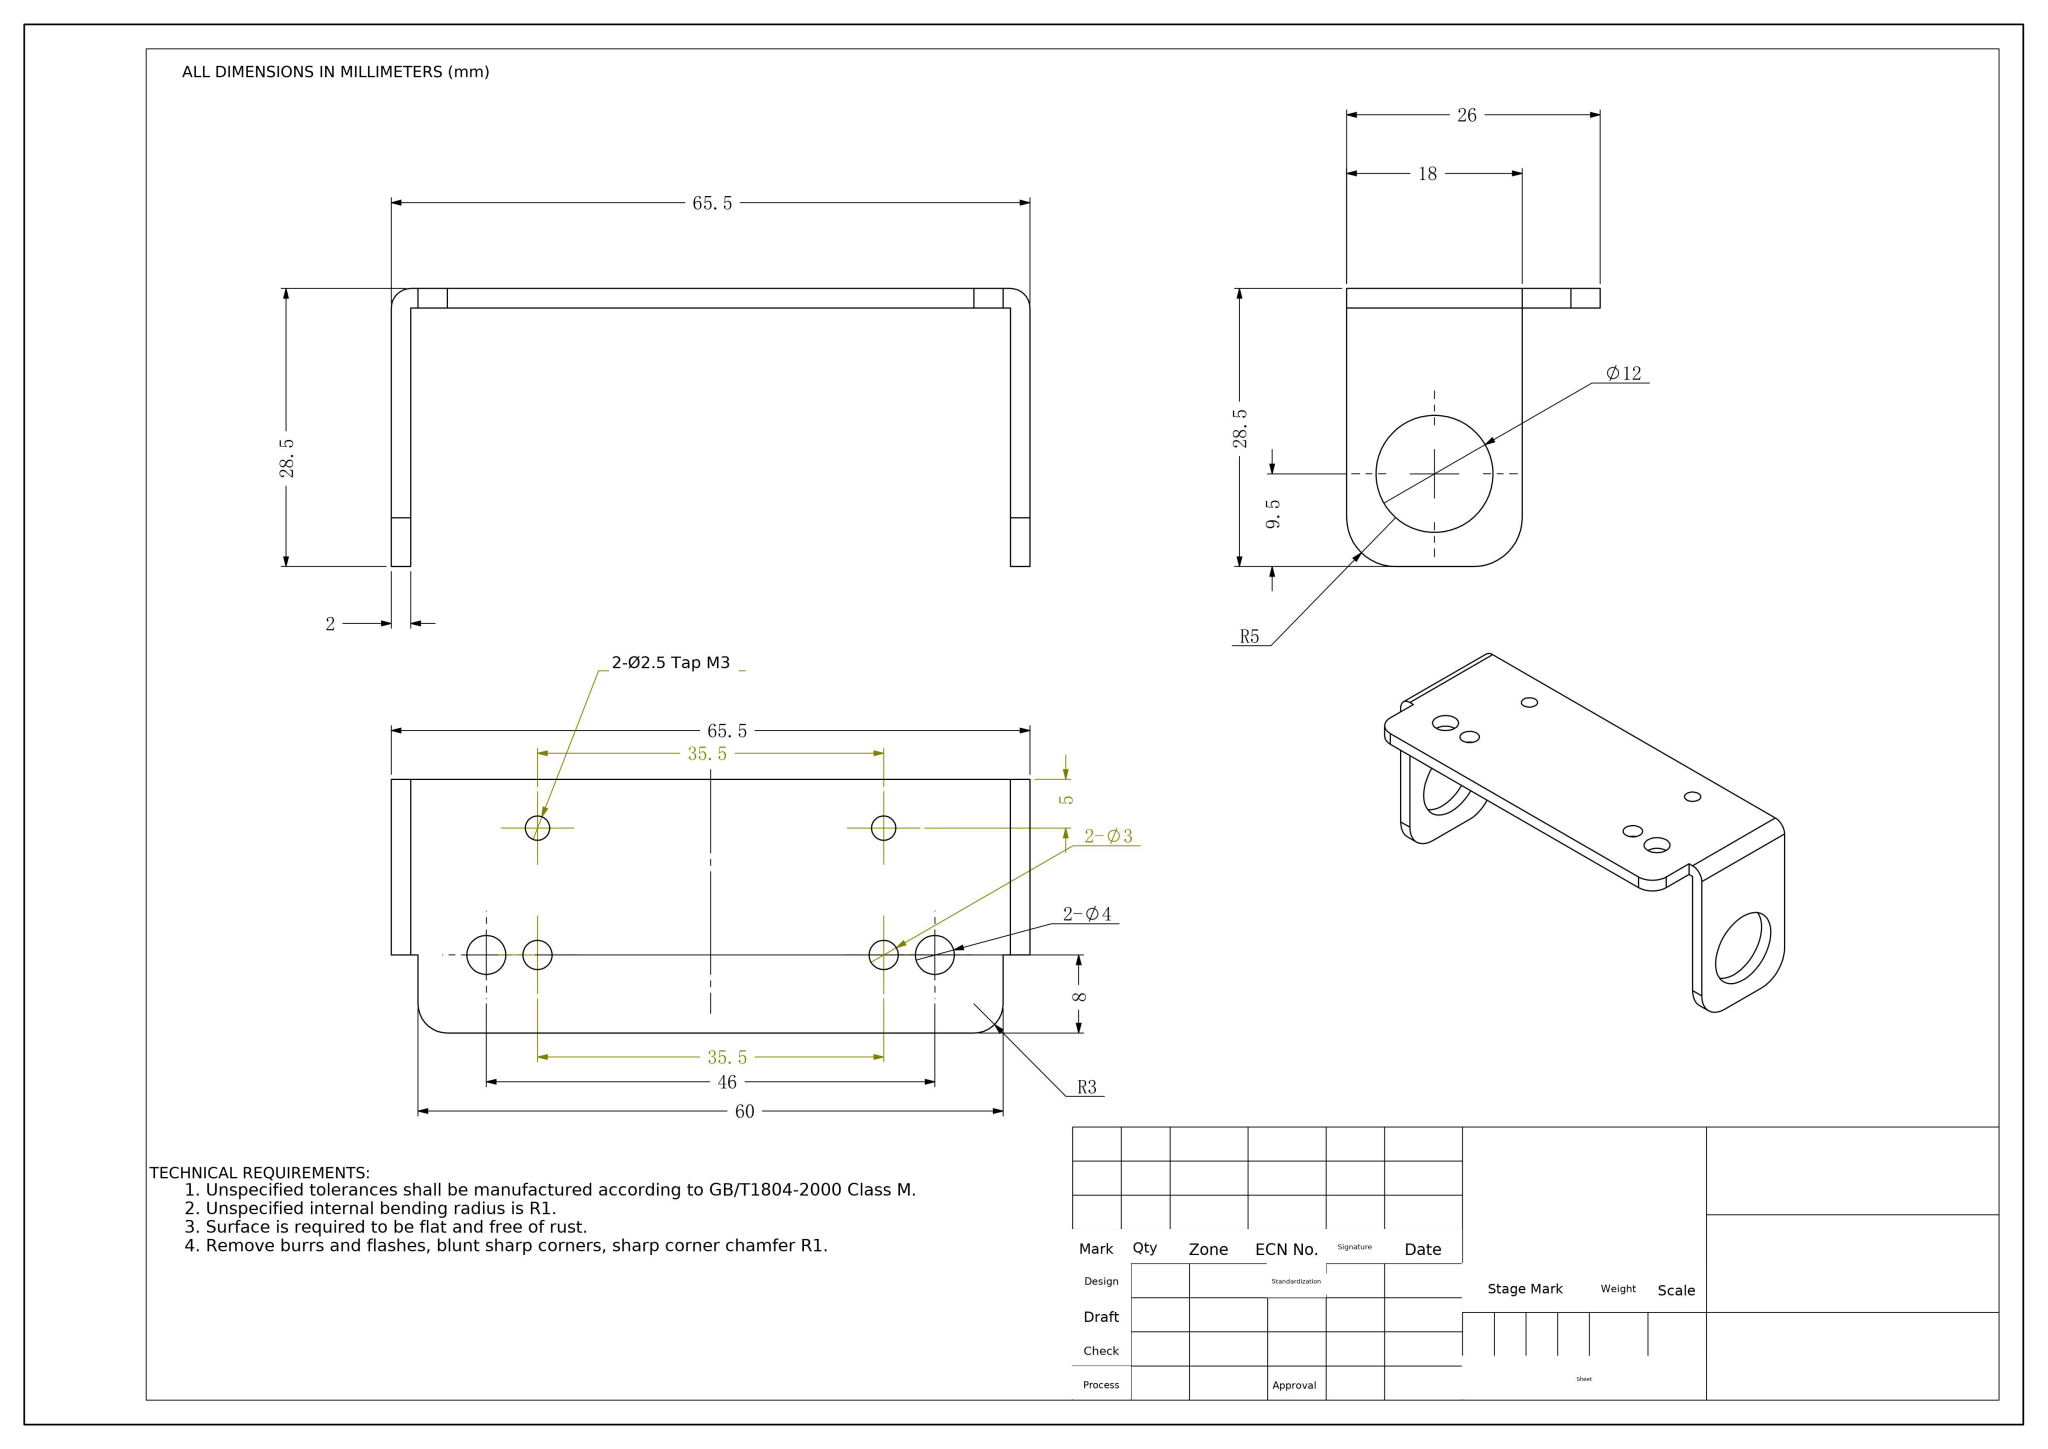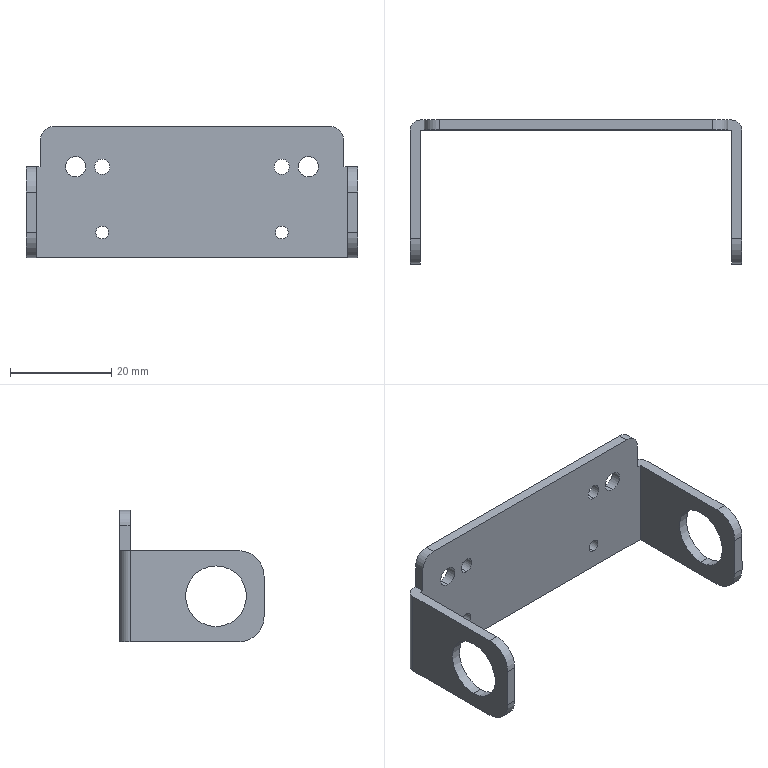Part | NX | mm | 1 solid | 38 faces | box 65.5 x 28.5 x 26 mm | volume 4594 mm3 | cylinder 24 | plane 14 | commonest cylinder face diameters 2.5 x4 4 x4 3 x4 12 x4 10 x4 4.004 x2 6 x2